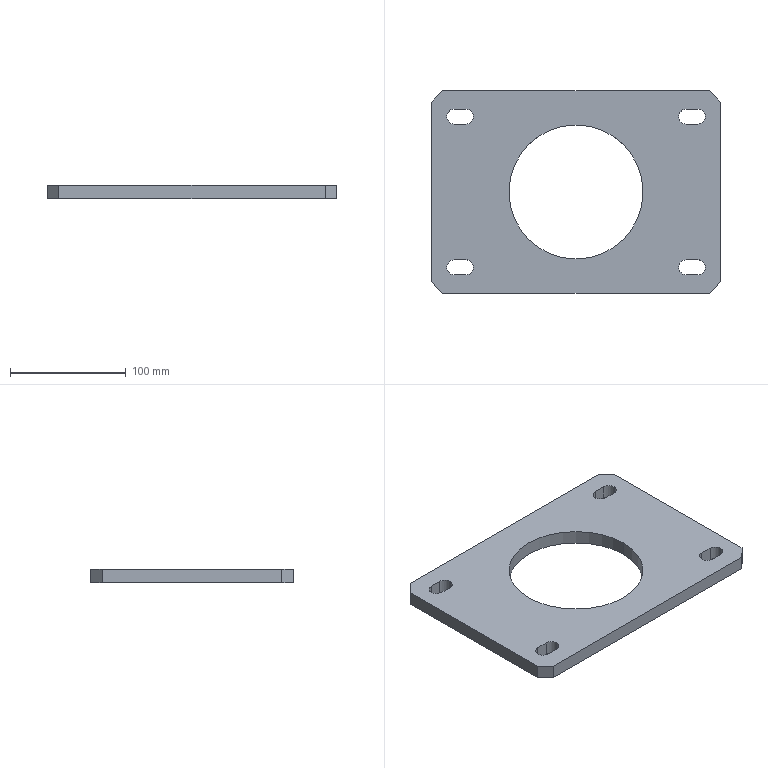Component | SolidWorks | PlanetaryReducer-PLF142Mount1-1 | 1 solid | 32 faces | box 250 x 175 x 12 mm | volume 384260 mm3 | plane 18 | cylinder 14 | commonest cylinder face diameters 13 x12 115.5 x2
build123d program:
from build123d import *

# Parameters (mm, degrees)
SKETCH1_W           = 250
SKETCH1_H           = 175
BOSS_EXTRUDE1_DEPTH = 12
SKETCH2_R           = 57.75
CUT_EXTRUDE1_DEPTH  = 154.053
CHAMFER1_SIZE       = 10
CUT_EXTRUDE2_DEPTH  = 154.053


with BuildPart() as part:
    # Sketch1 → Boss-Extrude1 (new body)
    with BuildSketch(Plane.XY):
        Rectangle(SKETCH1_W, SKETCH1_H)
    extrude(amount=BOSS_EXTRUDE1_DEPTH)

    # Sketch2 → Cut-Extrude1 (cut, through all)
    with BuildSketch(Plane.XY.offset(12)):
        Circle(SKETCH2_R)
    extrude(amount=-CUT_EXTRUDE1_DEPTH, mode=Mode.SUBTRACT)

    # Chamfer1
    chamfer1_edges = [part.edges().sort_by_distance(p)[0] for p in [
        (125, -87.5, 6),
        (-125, -87.5, 6),
        (-125, 87.5, 6),
        (125, 87.5, 6),
    ]]
    chamfer(chamfer1_edges, length=CHAMFER1_SIZE)

    # Sketch3 → Cut-Extrude2 (cut, through all)
    with BuildSketch(Plane.XY.offset(12)):
        with BuildLine():
            Line((-105, 71.5), (-95, 71.5))
            ThreePointArc((-95, 71.5), (-88.5, 65), (-95, 58.5))
            Line((-95, 58.5), (-105, 58.5))
            ThreePointArc((-105, 58.5), (-111.5, 65), (-105, 71.5))
        make_face()
        with BuildLine():
            Line((-105, -58.5), (-95, -58.5))
            ThreePointArc((-95, -58.5), (-88.5, -65), (-95, -71.5))
            Line((-95, -71.5), (-105, -71.5))
            ThreePointArc((-105, -71.5), (-111.5, -65), (-105, -58.5))
        make_face()
        with BuildLine():
            Line((95, -58.5), (105, -58.5))
            ThreePointArc((105, -58.5), (111.5, -65), (105, -71.5))
            Line((105, -71.5), (95, -71.5))
            ThreePointArc((95, -71.5), (88.5, -65), (95, -58.5))
        make_face()
        with BuildLine():
            Line((95, 71.5), (105, 71.5))
            ThreePointArc((105, 71.5), (111.5, 65), (105, 58.5))
            Line((105, 58.5), (95, 58.5))
            ThreePointArc((95, 58.5), (88.5, 65), (95, 71.5))
        make_face()
    extrude(amount=-CUT_EXTRUDE2_DEPTH, mode=Mode.SUBTRACT)


solid = part.part

# Placed as in the assembly
solid = solid.moved(Location((-85, 178, 110), (0, 0, 0)))
STEP:
#1=COLOUR_RGB('',0.7922,0.8196,0.9333);
#2=FILL_AREA_STYLE_COLOUR('',#1);
#3=FILL_AREA_STYLE('',(#2));
#4=SURFACE_STYLE_FILL_AREA(#3);
#5=SURFACE_SIDE_STYLE('',(#4));
#6=SURFACE_STYLE_USAGE(.BOTH.,#5);
#7=PRESENTATION_STYLE_ASSIGNMENT((#6));
#8=CARTESIAN_POINT('',(1.043,9.567,4.331));
#9=VERTEX_POINT('',#8);
#10=CARTESIAN_POINT('',(0.7874,9.823,4.331));
#11=VERTEX_POINT('',#10);
#12=CARTESIAN_POINT('',(0.7874,9.567,4.331));
#13=DIRECTION('',(0.,0.,1.));
#14=DIRECTION('',(1.,0.,0.));
#15=AXIS2_PLACEMENT_3D('',#12,#13,#14);
#16=CIRCLE('',#15,0.2559);
#17=EDGE_CURVE('',#9,#11,#16,.T.);
#18=ORIENTED_EDGE('',*,*,#17,.F.);
#19=CARTESIAN_POINT('',(1.043,9.567,4.803));
#20=VERTEX_POINT('',#19);
#21=CARTESIAN_POINT('',(1.043,9.567,4.331));
#22=DIRECTION('',(0.,0.,1.));
#23=VECTOR('',#22,39.37);
#24=LINE('',#21,#23);
#25=EDGE_CURVE('',#9,#20,#24,.T.);
#26=ORIENTED_EDGE('',*,*,#25,.T.);
#27=CARTESIAN_POINT('',(0.7874,9.823,4.803));
#28=VERTEX_POINT('',#27);
#29=CARTESIAN_POINT('',(0.7874,9.567,4.803));
#30=DIRECTION('',(0.,0.,1.));
#31=DIRECTION('',(1.,0.,0.));
#32=AXIS2_PLACEMENT_3D('',#29,#30,#31);
#33=CIRCLE('',#32,0.2559);
#34=EDGE_CURVE('',#20,#28,#33,.T.);
#35=ORIENTED_EDGE('',*,*,#34,.T.);
#36=CARTESIAN_POINT('',(0.7874,9.823,4.331));
#37=DIRECTION('',(0.,0.,1.));
#38=VECTOR('',#37,39.37);
#39=LINE('',#36,#38);
#40=EDGE_CURVE('',#11,#28,#39,.T.);
#41=ORIENTED_EDGE('',*,*,#40,.F.);
#42=EDGE_LOOP('',(#18,#26,#35,#41));
#43=FACE_OUTER_BOUND('',#42,.T.);
#44=CARTESIAN_POINT('',(0.7874,9.567,4.331));
#45=DIRECTION('',(0.,0.,1.));
#46=DIRECTION('',(1.,0.,0.));
#47=AXIS2_PLACEMENT_3D('',#44,#45,#46);
#48=CYLINDRICAL_SURFACE('',#47,0.2559);
#49=ADVANCED_FACE('',(#43),#48,.F.);
#50=CARTESIAN_POINT('',(1.043,4.449,4.331));
#51=VERTEX_POINT('',#50);
#52=CARTESIAN_POINT('',(0.7874,4.705,4.331));
#53=VERTEX_POINT('',#52);
#54=CARTESIAN_POINT('',(0.7874,4.449,4.331));
#55=DIRECTION('',(0.,0.,1.));
#56=DIRECTION('',(1.,0.,0.));
#57=AXIS2_PLACEMENT_3D('',#54,#55,#56);
#58=CIRCLE('',#57,0.2559);
#59=EDGE_CURVE('',#51,#53,#58,.T.);
#60=ORIENTED_EDGE('',*,*,#59,.F.);
#61=CARTESIAN_POINT('',(1.043,4.449,4.803));
#62=VERTEX_POINT('',#61);
#63=CARTESIAN_POINT('',(1.043,4.449,4.331));
#64=DIRECTION('',(0.,0.,1.));
#65=VECTOR('',#64,39.37);
#66=LINE('',#63,#65);
#67=EDGE_CURVE('',#51,#62,#66,.T.);
#68=ORIENTED_EDGE('',*,*,#67,.T.);
#69=CARTESIAN_POINT('',(0.7874,4.705,4.803));
#70=VERTEX_POINT('',#69);
#71=CARTESIAN_POINT('',(0.7874,4.449,4.803));
#72=DIRECTION('',(0.,0.,1.));
#73=DIRECTION('',(1.,0.,0.));
#74=AXIS2_PLACEMENT_3D('',#71,#72,#73);
#75=CIRCLE('',#74,0.2559);
#76=EDGE_CURVE('',#62,#70,#75,.T.);
#77=ORIENTED_EDGE('',*,*,#76,.T.);
#78=CARTESIAN_POINT('',(0.7874,4.705,4.331));
#79=DIRECTION('',(0.,0.,1.));
#80=VECTOR('',#79,39.37);
#81=LINE('',#78,#80);
#82=EDGE_CURVE('',#53,#70,#81,.T.);
#83=ORIENTED_EDGE('',*,*,#82,.F.);
#84=EDGE_LOOP('',(#60,#68,#77,#83));
#85=FACE_OUTER_BOUND('',#84,.T.);
#86=CARTESIAN_POINT('',(0.7874,4.449,4.331));
#87=DIRECTION('',(0.,0.,1.));
#88=DIRECTION('',(1.,0.,0.));
#89=AXIS2_PLACEMENT_3D('',#86,#87,#88);
#90=CYLINDRICAL_SURFACE('',#89,0.2559);
#91=ADVANCED_FACE('',(#85),#90,.F.);
#92=CARTESIAN_POINT('',(-6.831,4.449,4.331));
#93=VERTEX_POINT('',#92);
#94=CARTESIAN_POINT('',(-7.087,4.705,4.331));
#95=VERTEX_POINT('',#94);
#96=CARTESIAN_POINT('',(-7.087,4.449,4.331));
#97=DIRECTION('',(0.,0.,1.));
#98=DIRECTION('',(1.,0.,0.));
#99=AXIS2_PLACEMENT_3D('',#96,#97,#98);
#100=CIRCLE('',#99,0.2559);
#101=EDGE_CURVE('',#93,#95,#100,.T.);
#102=ORIENTED_EDGE('',*,*,#101,.F.);
#103=CARTESIAN_POINT('',(-6.831,4.449,4.803));
#104=VERTEX_POINT('',#103);
#105=CARTESIAN_POINT('',(-6.831,4.449,4.331));
#106=DIRECTION('',(0.,0.,1.));
#107=VECTOR('',#106,39.37);
#108=LINE('',#105,#107);
#109=EDGE_CURVE('',#93,#104,#108,.T.);
#110=ORIENTED_EDGE('',*,*,#109,.T.);
#111=CARTESIAN_POINT('',(-7.087,4.705,4.803));
#112=VERTEX_POINT('',#111);
#113=CARTESIAN_POINT('',(-7.087,4.449,4.803));
#114=DIRECTION('',(0.,0.,1.));
#115=DIRECTION('',(1.,0.,0.));
#116=AXIS2_PLACEMENT_3D('',#113,#114,#115);
#117=CIRCLE('',#116,0.2559);
#118=EDGE_CURVE('',#104,#112,#117,.T.);
#119=ORIENTED_EDGE('',*,*,#118,.T.);
#120=CARTESIAN_POINT('',(-7.087,4.705,4.331));
#121=DIRECTION('',(0.,0.,1.));
#122=VECTOR('',#121,39.37);
#123=LINE('',#120,#122);
#124=EDGE_CURVE('',#95,#112,#123,.T.);
#125=ORIENTED_EDGE('',*,*,#124,.F.);
#126=EDGE_LOOP('',(#102,#110,#119,#125));
#127=FACE_OUTER_BOUND('',#126,.T.);
#128=CARTESIAN_POINT('',(-7.087,4.449,4.331));
#129=DIRECTION('',(0.,0.,1.));
#130=DIRECTION('',(1.,0.,0.));
#131=AXIS2_PLACEMENT_3D('',#128,#129,#130);
#132=CYLINDRICAL_SURFACE('',#131,0.2559);
#133=ADVANCED_FACE('',(#127),#132,.F.);
#134=CARTESIAN_POINT('',(-6.831,9.567,4.331));
#135=VERTEX_POINT('',#134);
#136=CARTESIAN_POINT('',(-7.087,9.823,4.331));
#137=VERTEX_POINT('',#136);
#138=CARTESIAN_POINT('',(-7.087,9.567,4.331));
#139=DIRECTION('',(0.,0.,1.));
#140=DIRECTION('',(1.,0.,0.));
#141=AXIS2_PLACEMENT_3D('',#138,#139,#140);
#142=CIRCLE('',#141,0.2559);
#143=EDGE_CURVE('',#135,#137,#142,.T.);
#144=ORIENTED_EDGE('',*,*,#143,.F.);
#145=CARTESIAN_POINT('',(-6.831,9.567,4.803));
#146=VERTEX_POINT('',#145);
#147=CARTESIAN_POINT('',(-6.831,9.567,4.331));
#148=DIRECTION('',(0.,0.,1.));
#149=VECTOR('',#148,39.37);
#150=LINE('',#147,#149);
#151=EDGE_CURVE('',#135,#146,#150,.T.);
#152=ORIENTED_EDGE('',*,*,#151,.T.);
#153=CARTESIAN_POINT('',(-7.087,9.823,4.803));
#154=VERTEX_POINT('',#153);
#155=CARTESIAN_POINT('',(-7.087,9.567,4.803));
#156=DIRECTION('',(0.,0.,1.));
#157=DIRECTION('',(1.,0.,0.));
#158=AXIS2_PLACEMENT_3D('',#155,#156,#157);
#159=CIRCLE('',#158,0.2559);
#160=EDGE_CURVE('',#146,#154,#159,.T.);
#161=ORIENTED_EDGE('',*,*,#160,.T.);
#162=CARTESIAN_POINT('',(-7.087,9.823,4.331));
#163=DIRECTION('',(0.,0.,1.));
#164=VECTOR('',#163,39.37);
#165=LINE('',#162,#164);
#166=EDGE_CURVE('',#137,#154,#165,.T.);
#167=ORIENTED_EDGE('',*,*,#166,.F.);
#168=EDGE_LOOP('',(#144,#152,#161,#167));
#169=FACE_OUTER_BOUND('',#168,.T.);
#170=CARTESIAN_POINT('',(-7.087,9.567,4.331));
#171=DIRECTION('',(0.,0.,1.));
#172=DIRECTION('',(1.,0.,0.));
#173=AXIS2_PLACEMENT_3D('',#170,#171,#172);
#174=CYLINDRICAL_SURFACE('',#173,0.2559);
#175=ADVANCED_FACE('',(#169),#174,.F.);
#176=CARTESIAN_POINT('',(-5.62,7.008,4.331));
#177=VERTEX_POINT('',#176);
#178=CARTESIAN_POINT('',(-1.073,7.008,4.331));
#179=VERTEX_POINT('',#178);
#180=CARTESIAN_POINT('',(-3.346,7.008,4.331));
#181=DIRECTION('',(0.,0.,1.));
#182=DIRECTION('',(1.,0.,0.));
#183=AXIS2_PLACEMENT_3D('',#180,#181,#182);
#184=CIRCLE('',#183,2.274);
#185=EDGE_CURVE('',#177,#179,#184,.T.);
#186=ORIENTED_EDGE('',*,*,#185,.F.);
#187=CARTESIAN_POINT('',(-5.62,7.008,4.803));
#188=VERTEX_POINT('',#187);
#189=CARTESIAN_POINT('',(-5.62,7.008,4.331));
#190=DIRECTION('',(0.,0.,1.));
#191=VECTOR('',#190,39.37);
#192=LINE('',#189,#191);
#193=EDGE_CURVE('',#177,#188,#192,.T.);
#194=ORIENTED_EDGE('',*,*,#193,.T.);
#195=CARTESIAN_POINT('',(-1.073,7.008,4.803));
#196=VERTEX_POINT('',#195);
#197=CARTESIAN_POINT('',(-3.346,7.008,4.803));
#198=DIRECTION('',(0.,0.,1.));
#199=DIRECTION('',(1.,0.,0.));
#200=AXIS2_PLACEMENT_3D('',#197,#198,#199);
#201=CIRCLE('',#200,2.274);
#202=EDGE_CURVE('',#188,#196,#201,.T.);
#203=ORIENTED_EDGE('',*,*,#202,.T.);
#204=CARTESIAN_POINT('',(-1.073,7.008,4.331));
#205=DIRECTION('',(0.,0.,1.));
#206=VECTOR('',#205,39.37);
#207=LINE('',#204,#206);
#208=EDGE_CURVE('',#179,#196,#207,.T.);
#209=ORIENTED_EDGE('',*,*,#208,.F.);
#210=EDGE_LOOP('',(#186,#194,#203,#209));
#211=FACE_OUTER_BOUND('',#210,.T.);
#212=CARTESIAN_POINT('',(-3.346,7.008,4.331));
#213=DIRECTION('',(0.,0.,1.));
#214=DIRECTION('',(1.,0.,0.));
#215=AXIS2_PLACEMENT_3D('',#212,#213,#214);
#216=CYLINDRICAL_SURFACE('',#215,2.274);
#217=ADVANCED_FACE('',(#211),#216,.F.);
#218=CARTESIAN_POINT('',(1.575,3.957,4.803));
#219=VERTEX_POINT('',#218);
#220=CARTESIAN_POINT('',(1.575,10.059,4.803));
#221=VERTEX_POINT('',#220);
#222=CARTESIAN_POINT('',(1.575,10.453,4.803));
#223=DIRECTION('',(-0.,1.,0.));
#224=VECTOR('',#223,39.37);
#225=LINE('',#222,#224);
#226=EDGE_CURVE('',#219,#221,#225,.T.);
#227=ORIENTED_EDGE('',*,*,#226,.F.);
#228=CARTESIAN_POINT('',(1.575,3.957,4.331));
#229=VERTEX_POINT('',#228);
#230=CARTESIAN_POINT('',(1.575,3.957,4.803));
#231=DIRECTION('',(0.,0.,-1.));
#232=VECTOR('',#231,39.37);
#233=LINE('',#230,#232);
#234=EDGE_CURVE('',#219,#229,#233,.T.);
#235=ORIENTED_EDGE('',*,*,#234,.T.);
#236=CARTESIAN_POINT('',(1.575,10.059,4.331));
#237=VERTEX_POINT('',#236);
#238=CARTESIAN_POINT('',(1.575,10.453,4.331));
#239=DIRECTION('',(-0.,1.,0.));
#240=VECTOR('',#239,39.37);
#241=LINE('',#238,#240);
#242=EDGE_CURVE('',#229,#237,#241,.T.);
#243=ORIENTED_EDGE('',*,*,#242,.T.);
#244=CARTESIAN_POINT('',(1.575,10.059,4.803));
#245=DIRECTION('',(0.,0.,1.));
#246=VECTOR('',#245,39.37);
#247=LINE('',#244,#246);
#248=EDGE_CURVE('',#237,#221,#247,.T.);
#249=ORIENTED_EDGE('',*,*,#248,.T.);
#250=EDGE_LOOP('',(#227,#235,#243,#249));
#251=FACE_OUTER_BOUND('',#250,.T.);
#252=CARTESIAN_POINT('',(1.575,10.453,4.803));
#253=DIRECTION('',(-1.,-0.,0.));
#254=DIRECTION('',(0.,-1.,0.));
#255=AXIS2_PLACEMENT_3D('',#252,#253,#254);
#256=PLANE('',#255);
#257=ADVANCED_FACE('',(#251),#256,.F.);
#258=CARTESIAN_POINT('',(1.181,10.453,4.331));
#259=VERTEX_POINT('',#258);
#260=CARTESIAN_POINT('',(-7.874,10.453,4.331));
#261=VERTEX_POINT('',#260);
#262=CARTESIAN_POINT('',(-8.268,10.453,4.331));
#263=DIRECTION('',(-1.,0.,0.));
#264=VECTOR('',#263,39.37);
#265=LINE('',#262,#264);
#266=EDGE_CURVE('',#259,#261,#265,.T.);
#267=ORIENTED_EDGE('',*,*,#266,.T.);
#268=CARTESIAN_POINT('',(-7.874,10.453,4.803));
#269=VERTEX_POINT('',#268);
#270=CARTESIAN_POINT('',(-7.874,10.453,4.803));
#271=DIRECTION('',(0.,0.,1.));
#272=VECTOR('',#271,39.37);
#273=LINE('',#270,#272);
#274=EDGE_CURVE('',#261,#269,#273,.T.);
#275=ORIENTED_EDGE('',*,*,#274,.T.);
#276=CARTESIAN_POINT('',(1.181,10.453,4.803));
#277=VERTEX_POINT('',#276);
#278=CARTESIAN_POINT('',(-8.268,10.453,4.803));
#279=DIRECTION('',(-1.,0.,0.));
#280=VECTOR('',#279,39.37);
#281=LINE('',#278,#280);
#282=EDGE_CURVE('',#277,#269,#281,.T.);
#283=ORIENTED_EDGE('',*,*,#282,.F.);
#284=CARTESIAN_POINT('',(1.181,10.453,4.803));
#285=DIRECTION('',(0.,0.,-1.));
#286=VECTOR('',#285,39.37);
#287=LINE('',#284,#286);
#288=EDGE_CURVE('',#277,#259,#287,.T.);
#289=ORIENTED_EDGE('',*,*,#288,.T.);
#290=EDGE_LOOP('',(#267,#275,#283,#289));
#291=FACE_OUTER_BOUND('',#290,.T.);
#292=CARTESIAN_POINT('',(-8.268,10.453,4.803));
#293=DIRECTION('',(0.,-1.,0.));
#294=DIRECTION('',(0.,0.,-1.));
#295=AXIS2_PLACEMENT_3D('',#292,#293,#294);
#296=PLANE('',#295);
#297=ADVANCED_FACE('',(#291),#296,.F.);
#298=CARTESIAN_POINT('',(-8.268,10.059,4.331));
#299=VERTEX_POINT('',#298);
#300=CARTESIAN_POINT('',(-8.268,3.957,4.331));
#301=VERTEX_POINT('',#300);
#302=CARTESIAN_POINT('',(-8.268,10.453,4.331));
#303=DIRECTION('',(0.,-1.,0.));
#304=VECTOR('',#303,39.37);
#305=LINE('',#302,#304);
#306=EDGE_CURVE('',#299,#301,#305,.T.);
#307=ORIENTED_EDGE('',*,*,#306,.T.);
#308=CARTESIAN_POINT('',(-8.268,3.957,4.803));
#309=VERTEX_POINT('',#308);
#310=CARTESIAN_POINT('',(-8.268,3.957,4.803));
#311=DIRECTION('',(0.,0.,1.));
#312=VECTOR('',#311,39.37);
#313=LINE('',#310,#312);
#314=EDGE_CURVE('',#301,#309,#313,.T.);
#315=ORIENTED_EDGE('',*,*,#314,.T.);
#316=CARTESIAN_POINT('',(-8.268,10.059,4.803));
#317=VERTEX_POINT('',#316);
#318=CARTESIAN_POINT('',(-8.268,10.453,4.803));
#319=DIRECTION('',(0.,-1.,0.));
#320=VECTOR('',#319,39.37);
#321=LINE('',#318,#320);
#322=EDGE_CURVE('',#317,#309,#321,.T.);
#323=ORIENTED_EDGE('',*,*,#322,.F.);
#324=CARTESIAN_POINT('',(-8.268,10.059,4.803));
#325=DIRECTION('',(0.,0.,-1.));
#326=VECTOR('',#325,39.37);
#327=LINE('',#324,#326);
#328=EDGE_CURVE('',#317,#299,#327,.T.);
#329=ORIENTED_EDGE('',*,*,#328,.T.);
#330=EDGE_LOOP('',(#307,#315,#323,#329));
#331=FACE_OUTER_BOUND('',#330,.T.);
#332=CARTESIAN_POINT('',(-8.268,10.453,4.803));
#333=DIRECTION('',(1.,0.,0.));
#334=DIRECTION('',(-0.,1.,0.));
#335=AXIS2_PLACEMENT_3D('',#332,#333,#334);
#336=PLANE('',#335);
#337=ADVANCED_FACE('',(#331),#336,.F.);
#338=CARTESIAN_POINT('',(-7.874,3.563,4.331));
#339=VERTEX_POINT('',#338);
#340=CARTESIAN_POINT('',(1.181,3.563,4.331));
#341=VERTEX_POINT('',#340);
#342=CARTESIAN_POINT('',(-8.268,3.563,4.331));
#343=DIRECTION('',(1.,0.,0.));
#344=VECTOR('',#343,39.37);
#345=LINE('',#342,#344);
#346=EDGE_CURVE('',#339,#341,#345,.T.);
#347=ORIENTED_EDGE('',*,*,#346,.T.);
#348=CARTESIAN_POINT('',(1.181,3.563,4.803));
#349=VERTEX_POINT('',#348);
#350=CARTESIAN_POINT('',(1.181,3.563,4.803));
#351=DIRECTION('',(0.,0.,1.));
#352=VECTOR('',#351,39.37);
#353=LINE('',#350,#352);
#354=EDGE_CURVE('',#341,#349,#353,.T.);
#355=ORIENTED_EDGE('',*,*,#354,.T.);
#356=CARTESIAN_POINT('',(-7.874,3.563,4.803));
#357=VERTEX_POINT('',#356);
#358=CARTESIAN_POINT('',(-8.268,3.563,4.803));
#359=DIRECTION('',(1.,0.,0.));
#360=VECTOR('',#359,39.37);
#361=LINE('',#358,#360);
#362=EDGE_CURVE('',#357,#349,#361,.T.);
#363=ORIENTED_EDGE('',*,*,#362,.F.);
#364=CARTESIAN_POINT('',(-7.874,3.563,4.803));
#365=DIRECTION('',(0.,0.,-1.));
#366=VECTOR('',#365,39.37);
#367=LINE('',#364,#366);
#368=EDGE_CURVE('',#357,#339,#367,.T.);
#369=ORIENTED_EDGE('',*,*,#368,.T.);
#370=EDGE_LOOP('',(#347,#355,#363,#369));
#371=FACE_OUTER_BOUND('',#370,.T.);
#372=CARTESIAN_POINT('',(-8.268,3.563,4.803));
#373=DIRECTION('',(0.,1.,0.));
#374=DIRECTION('',(0.,0.,1.));
#375=AXIS2_PLACEMENT_3D('',#372,#373,#374);
#376=PLANE('',#375);
#377=ADVANCED_FACE('',(#371),#376,.F.);
#378=CARTESIAN_POINT('',(0.3937,9.823,4.803));
#379=VERTEX_POINT('',#378);
#380=CARTESIAN_POINT('',(0.3937,9.311,4.803));
#381=VERTEX_POINT('',#380);
#382=CARTESIAN_POINT('',(0.3937,9.567,4.803));
#383=DIRECTION('',(0.,0.,1.));
#384=DIRECTION('',(1.,0.,0.));
#385=AXIS2_PLACEMENT_3D('',#382,#383,#384);
#386=CIRCLE('',#385,0.2559);
#387=EDGE_CURVE('',#379,#381,#386,.T.);
#388=ORIENTED_EDGE('',*,*,#387,.F.);
#389=CARTESIAN_POINT('',(0.3937,9.823,4.803));
#390=DIRECTION('',(-1.,0.,0.));
#391=VECTOR('',#390,39.37);
#392=LINE('',#389,#391);
#393=EDGE_CURVE('',#28,#379,#392,.T.);
#394=ORIENTED_EDGE('',*,*,#393,.F.);
#395=ORIENTED_EDGE('',*,*,#34,.F.);
#396=CARTESIAN_POINT('',(0.7874,9.311,4.803));
#397=VERTEX_POINT('',#396);
#398=CARTESIAN_POINT('',(0.7874,9.567,4.803));
#399=DIRECTION('',(0.,0.,1.));
#400=DIRECTION('',(1.,0.,0.));
#401=AXIS2_PLACEMENT_3D('',#398,#399,#400);
#402=CIRCLE('',#401,0.2559);
#403=EDGE_CURVE('',#397,#20,#402,.T.);
#404=ORIENTED_EDGE('',*,*,#403,.F.);
#405=CARTESIAN_POINT('',(0.3937,9.311,4.803));
#406=DIRECTION('',(1.,0.,0.));
#407=VECTOR('',#406,39.37);
#408=LINE('',#405,#407);
#409=EDGE_CURVE('',#381,#397,#408,.T.);
#410=ORIENTED_EDGE('',*,*,#409,.F.);
#411=EDGE_LOOP('',(#388,#394,#395,#404,#410));
#412=FACE_BOUND('',#411,.T.);
#413=CARTESIAN_POINT('',(0.3937,4.705,4.803));
#414=VERTEX_POINT('',#413);
#415=CARTESIAN_POINT('',(0.3937,4.193,4.803));
#416=VERTEX_POINT('',#415);
#417=CARTESIAN_POINT('',(0.3937,4.449,4.803));
#418=DIRECTION('',(0.,0.,1.));
#419=DIRECTION('',(1.,0.,0.));
#420=AXIS2_PLACEMENT_3D('',#417,#418,#419);
#421=CIRCLE('',#420,0.2559);
#422=EDGE_CURVE('',#414,#416,#421,.T.);
#423=ORIENTED_EDGE('',*,*,#422,.F.);
#424=CARTESIAN_POINT('',(0.3937,4.705,4.803));
#425=DIRECTION('',(-1.,0.,0.));
#426=VECTOR('',#425,39.37);
#427=LINE('',#424,#426);
#428=EDGE_CURVE('',#70,#414,#427,.T.);
#429=ORIENTED_EDGE('',*,*,#428,.F.);
#430=ORIENTED_EDGE('',*,*,#76,.F.);
#431=CARTESIAN_POINT('',(0.7874,4.193,4.803));
#432=VERTEX_POINT('',#431);
#433=CARTESIAN_POINT('',(0.7874,4.449,4.803));
#434=DIRECTION('',(0.,0.,1.));
#435=DIRECTION('',(1.,0.,0.));
#436=AXIS2_PLACEMENT_3D('',#433,#434,#435);
#437=CIRCLE('',#436,0.2559);
#438=EDGE_CURVE('',#432,#62,#437,.T.);
#439=ORIENTED_EDGE('',*,*,#438,.F.);
#440=CARTESIAN_POINT('',(0.3937,4.193,4.803));
#441=DIRECTION('',(1.,0.,0.));
#442=VECTOR('',#441,39.37);
#443=LINE('',#440,#442);
#444=EDGE_CURVE('',#416,#432,#443,.T.);
#445=ORIENTED_EDGE('',*,*,#444,.F.);
#446=EDGE_LOOP('',(#423,#429,#430,#439,#445));
#447=FACE_BOUND('',#446,.T.);
#448=CARTESIAN_POINT('',(-7.48,4.705,4.803));
#449=VERTEX_POINT('',#448);
#450=CARTESIAN_POINT('',(-7.48,4.193,4.803));
#451=VERTEX_POINT('',#450);
#452=CARTESIAN_POINT('',(-7.48,4.449,4.803));
#453=DIRECTION('',(0.,0.,1.));
#454=DIRECTION('',(1.,0.,0.));
#455=AXIS2_PLACEMENT_3D('',#452,#453,#454);
#456=CIRCLE('',#455,0.2559);
#457=EDGE_CURVE('',#449,#451,#456,.T.);
#458=ORIENTED_EDGE('',*,*,#457,.F.);
#459=CARTESIAN_POINT('',(-7.48,4.705,4.803));
#460=DIRECTION('',(-1.,0.,0.));
#461=VECTOR('',#460,39.37);
#462=LINE('',#459,#461);
#463=EDGE_CURVE('',#112,#449,#462,.T.);
#464=ORIENTED_EDGE('',*,*,#463,.F.);
#465=ORIENTED_EDGE('',*,*,#118,.F.);
#466=CARTESIAN_POINT('',(-7.087,4.193,4.803));
#467=VERTEX_POINT('',#466);
#468=CARTESIAN_POINT('',(-7.087,4.449,4.803));
#469=DIRECTION('',(0.,0.,1.));
#470=DIRECTION('',(1.,0.,0.));
#471=AXIS2_PLACEMENT_3D('',#468,#469,#470);
#472=CIRCLE('',#471,0.2559);
#473=EDGE_CURVE('',#467,#104,#472,.T.);
#474=ORIENTED_EDGE('',*,*,#473,.F.);
#475=CARTESIAN_POINT('',(-7.48,4.193,4.803));
#476=DIRECTION('',(1.,0.,0.));
#477=VECTOR('',#476,39.37);
#478=LINE('',#475,#477);
#479=EDGE_CURVE('',#451,#467,#478,.T.);
#480=ORIENTED_EDGE('',*,*,#479,.F.);
#481=EDGE_LOOP('',(#458,#464,#465,#474,#480));
#482=FACE_BOUND('',#481,.T.);
#483=CARTESIAN_POINT('',(-7.48,9.823,4.803));
#484=VERTEX_POINT('',#483);
#485=CARTESIAN_POINT('',(-7.48,9.311,4.803));
#486=VERTEX_POINT('',#485);
#487=CARTESIAN_POINT('',(-7.48,9.567,4.803));
#488=DIRECTION('',(0.,0.,1.));
#489=DIRECTION('',(1.,0.,0.));
#490=AXIS2_PLACEMENT_3D('',#487,#488,#489);
#491=CIRCLE('',#490,0.2559);
#492=EDGE_CURVE('',#484,#486,#491,.T.);
#493=ORIENTED_EDGE('',*,*,#492,.F.);
#494=CARTESIAN_POINT('',(-7.48,9.823,4.803));
#495=DIRECTION('',(-1.,0.,0.));
#496=VECTOR('',#495,39.37);
#497=LINE('',#494,#496);
#498=EDGE_CURVE('',#154,#484,#497,.T.);
#499=ORIENTED_EDGE('',*,*,#498,.F.);
#500=ORIENTED_EDGE('',*,*,#160,.F.);
#501=CARTESIAN_POINT('',(-7.087,9.311,4.803));
#502=VERTEX_POINT('',#501);
#503=CARTESIAN_POINT('',(-7.087,9.567,4.803));
#504=DIRECTION('',(0.,0.,1.));
#505=DIRECTION('',(1.,0.,0.));
#506=AXIS2_PLACEMENT_3D('',#503,#504,#505);
#507=CIRCLE('',#506,0.2559);
#508=EDGE_CURVE('',#502,#146,#507,.T.);
#509=ORIENTED_EDGE('',*,*,#508,.F.);
#510=CARTESIAN_POINT('',(-7.48,9.311,4.803));
#511=DIRECTION('',(1.,0.,0.));
#512=VECTOR('',#511,39.37);
#513=LINE('',#510,#512);
#514=EDGE_CURVE('',#486,#502,#513,.T.);
#515=ORIENTED_EDGE('',*,*,#514,.F.);
#516=EDGE_LOOP('',(#493,#499,#500,#509,#515));
#517=FACE_BOUND('',#516,.T.);
#518=CARTESIAN_POINT('',(-3.346,7.008,4.803));
#519=DIRECTION('',(0.,0.,1.));
#520=DIRECTION('',(1.,0.,0.));
#521=AXIS2_PLACEMENT_3D('',#518,#519,#520);
#522=CIRCLE('',#521,2.274);
#523=EDGE_CURVE('',#196,#188,#522,.T.);
#524=ORIENTED_EDGE('',*,*,#523,.F.);
#525=ORIENTED_EDGE('',*,*,#202,.F.);
#526=EDGE_LOOP('',(#524,#525));
#527=FACE_BOUND('',#526,.T.);
#528=ORIENTED_EDGE('',*,*,#362,.T.);
#529=CARTESIAN_POINT('',(0.6398,3.022,4.803));
#530=DIRECTION('',(0.7071,0.7071,0.));
#531=VECTOR('',#530,39.37);
#532=LINE('',#529,#531);
#533=EDGE_CURVE('',#349,#219,#532,.T.);
#534=ORIENTED_EDGE('',*,*,#533,.T.);
#535=ORIENTED_EDGE('',*,*,#226,.T.);
#536=CARTESIAN_POINT('',(0.6398,10.994,4.803));
#537=DIRECTION('',(-0.7071,0.7071,0.));
#538=VECTOR('',#537,39.37);
#539=LINE('',#536,#538);
#540=EDGE_CURVE('',#221,#277,#539,.T.);
#541=ORIENTED_EDGE('',*,*,#540,.T.);
#542=ORIENTED_EDGE('',*,*,#282,.T.);
#543=CARTESIAN_POINT('',(-7.333,10.994,4.803));
#544=DIRECTION('',(-0.7071,-0.7071,0.));
#545=VECTOR('',#544,39.37);
#546=LINE('',#543,#545);
#547=EDGE_CURVE('',#269,#317,#546,.T.);
#548=ORIENTED_EDGE('',*,*,#547,.T.);
#549=ORIENTED_EDGE('',*,*,#322,.T.);
#550=CARTESIAN_POINT('',(-7.333,3.022,4.803));
#551=DIRECTION('',(0.7071,-0.7071,0.));
#552=VECTOR('',#551,39.37);
#553=LINE('',#550,#552);
#554=EDGE_CURVE('',#309,#357,#553,.T.);
#555=ORIENTED_EDGE('',*,*,#554,.T.);
#556=EDGE_LOOP('',(#528,#534,#535,#541,#542,#548,#549,#555));
#557=FACE_OUTER_BOUND('',#556,.T.);
#558=CARTESIAN_POINT('',(-3.346,7.008,4.803));
#559=DIRECTION('',(0.,0.,1.));
#560=DIRECTION('',(1.,0.,0.));
#561=AXIS2_PLACEMENT_3D('',#558,#559,#560);
#562=PLANE('',#561);
#563=ADVANCED_FACE('',(#412,#447,#482,#517,#527,#557),#562,.T.);
#564=CARTESIAN_POINT('',(0.3937,9.823,4.331));
#565=VERTEX_POINT('',#564);
#566=CARTESIAN_POINT('',(0.3937,9.823,4.331));
#567=DIRECTION('',(-1.,0.,0.));
#568=VECTOR('',#567,39.37);
#569=LINE('',#566,#568);
#570=EDGE_CURVE('',#11,#565,#569,.T.);
#571=ORIENTED_EDGE('',*,*,#570,.T.);
#572=CARTESIAN_POINT('',(0.3937,9.311,4.331));
#573=VERTEX_POINT('',#572);
#574=CARTESIAN_POINT('',(0.3937,9.567,4.331));
#575=DIRECTION('',(0.,0.,1.));
#576=DIRECTION('',(1.,0.,0.));
#577=AXIS2_PLACEMENT_3D('',#574,#575,#576);
#578=CIRCLE('',#577,0.2559);
#579=EDGE_CURVE('',#565,#573,#578,.T.);
#580=ORIENTED_EDGE('',*,*,#579,.T.);
#581=CARTESIAN_POINT('',(0.7874,9.311,4.331));
#582=VERTEX_POINT('',#581);
#583=CARTESIAN_POINT('',(0.3937,9.311,4.331));
#584=DIRECTION('',(1.,0.,0.));
#585=VECTOR('',#584,39.37);
#586=LINE('',#583,#585);
#587=EDGE_CURVE('',#573,#582,#586,.T.);
#588=ORIENTED_EDGE('',*,*,#587,.T.);
#589=CARTESIAN_POINT('',(0.7874,9.567,4.331));
#590=DIRECTION('',(0.,0.,1.));
#591=DIRECTION('',(1.,0.,0.));
#592=AXIS2_PLACEMENT_3D('',#589,#590,#591);
#593=CIRCLE('',#592,0.2559);
#594=EDGE_CURVE('',#582,#9,#593,.T.);
#595=ORIENTED_EDGE('',*,*,#594,.T.);
#596=ORIENTED_EDGE('',*,*,#17,.T.);
#597=EDGE_LOOP('',(#571,#580,#588,#595,#596));
#598=FACE_BOUND('',#597,.T.);
#599=CARTESIAN_POINT('',(0.3937,4.705,4.331));
#600=VERTEX_POINT('',#599);
#601=CARTESIAN_POINT('',(0.3937,4.705,4.331));
#602=DIRECTION('',(-1.,0.,0.));
#603=VECTOR('',#602,39.37);
#604=LINE('',#601,#603);
#605=EDGE_CURVE('',#53,#600,#604,.T.);
#606=ORIENTED_EDGE('',*,*,#605,.T.);
#607=CARTESIAN_POINT('',(0.3937,4.193,4.331));
#608=VERTEX_POINT('',#607);
#609=CARTESIAN_POINT('',(0.3937,4.449,4.331));
#610=DIRECTION('',(0.,0.,1.));
#611=DIRECTION('',(1.,0.,0.));
#612=AXIS2_PLACEMENT_3D('',#609,#610,#611);
#613=CIRCLE('',#612,0.2559);
#614=EDGE_CURVE('',#600,#608,#613,.T.);
#615=ORIENTED_EDGE('',*,*,#614,.T.);
#616=CARTESIAN_POINT('',(0.7874,4.193,4.331));
#617=VERTEX_POINT('',#616);
#618=CARTESIAN_POINT('',(0.3937,4.193,4.331));
#619=DIRECTION('',(1.,0.,0.));
#620=VECTOR('',#619,39.37);
#621=LINE('',#618,#620);
#622=EDGE_CURVE('',#608,#617,#621,.T.);
#623=ORIENTED_EDGE('',*,*,#622,.T.);
#624=CARTESIAN_POINT('',(0.7874,4.449,4.331));
#625=DIRECTION('',(0.,0.,1.));
#626=DIRECTION('',(1.,0.,0.));
#627=AXIS2_PLACEMENT_3D('',#624,#625,#626);
#628=CIRCLE('',#627,0.2559);
#629=EDGE_CURVE('',#617,#51,#628,.T.);
#630=ORIENTED_EDGE('',*,*,#629,.T.);
#631=ORIENTED_EDGE('',*,*,#59,.T.);
#632=EDGE_LOOP('',(#606,#615,#623,#630,#631));
#633=FACE_BOUND('',#632,.T.);
#634=CARTESIAN_POINT('',(-7.48,4.705,4.331));
#635=VERTEX_POINT('',#634);
#636=CARTESIAN_POINT('',(-7.48,4.705,4.331));
#637=DIRECTION('',(-1.,0.,0.));
#638=VECTOR('',#637,39.37);
#639=LINE('',#636,#638);
#640=EDGE_CURVE('',#95,#635,#639,.T.);
#641=ORIENTED_EDGE('',*,*,#640,.T.);
#642=CARTESIAN_POINT('',(-7.48,4.193,4.331));
#643=VERTEX_POINT('',#642);
#644=CARTESIAN_POINT('',(-7.48,4.449,4.331));
#645=DIRECTION('',(0.,0.,1.));
#646=DIRECTION('',(1.,0.,0.));
#647=AXIS2_PLACEMENT_3D('',#644,#645,#646);
#648=CIRCLE('',#647,0.2559);
#649=EDGE_CURVE('',#635,#643,#648,.T.);
#650=ORIENTED_EDGE('',*,*,#649,.T.);
#651=CARTESIAN_POINT('',(-7.087,4.193,4.331));
#652=VERTEX_POINT('',#651);
#653=CARTESIAN_POINT('',(-7.48,4.193,4.331));
#654=DIRECTION('',(1.,0.,0.));
#655=VECTOR('',#654,39.37);
#656=LINE('',#653,#655);
#657=EDGE_CURVE('',#643,#652,#656,.T.);
#658=ORIENTED_EDGE('',*,*,#657,.T.);
#659=CARTESIAN_POINT('',(-7.087,4.449,4.331));
#660=DIRECTION('',(0.,0.,1.));
#661=DIRECTION('',(1.,0.,0.));
#662=AXIS2_PLACEMENT_3D('',#659,#660,#661);
#663=CIRCLE('',#662,0.2559);
#664=EDGE_CURVE('',#652,#93,#663,.T.);
#665=ORIENTED_EDGE('',*,*,#664,.T.);
#666=ORIENTED_EDGE('',*,*,#101,.T.);
#667=EDGE_LOOP('',(#641,#650,#658,#665,#666));
#668=FACE_BOUND('',#667,.T.);
#669=CARTESIAN_POINT('',(-7.48,9.823,4.331));
#670=VERTEX_POINT('',#669);
#671=CARTESIAN_POINT('',(-7.48,9.823,4.331));
#672=DIRECTION('',(-1.,0.,0.));
#673=VECTOR('',#672,39.37);
#674=LINE('',#671,#673);
#675=EDGE_CURVE('',#137,#670,#674,.T.);
#676=ORIENTED_EDGE('',*,*,#675,.T.);
#677=CARTESIAN_POINT('',(-7.48,9.311,4.331));
#678=VERTEX_POINT('',#677);
#679=CARTESIAN_POINT('',(-7.48,9.567,4.331));
#680=DIRECTION('',(0.,0.,1.));
#681=DIRECTION('',(1.,0.,0.));
#682=AXIS2_PLACEMENT_3D('',#679,#680,#681);
#683=CIRCLE('',#682,0.2559);
#684=EDGE_CURVE('',#670,#678,#683,.T.);
#685=ORIENTED_EDGE('',*,*,#684,.T.);
#686=CARTESIAN_POINT('',(-7.087,9.311,4.331));
#687=VERTEX_POINT('',#686);
#688=CARTESIAN_POINT('',(-7.48,9.311,4.331));
#689=DIRECTION('',(1.,0.,0.));
#690=VECTOR('',#689,39.37);
#691=LINE('',#688,#690);
#692=EDGE_CURVE('',#678,#687,#691,.T.);
#693=ORIENTED_EDGE('',*,*,#692,.T.);
#694=CARTESIAN_POINT('',(-7.087,9.567,4.331));
#695=DIRECTION('',(0.,0.,1.));
#696=DIRECTION('',(1.,0.,0.));
#697=AXIS2_PLACEMENT_3D('',#694,#695,#696);
#698=CIRCLE('',#697,0.2559);
#699=EDGE_CURVE('',#687,#135,#698,.T.);
#700=ORIENTED_EDGE('',*,*,#699,.T.);
#701=ORIENTED_EDGE('',*,*,#143,.T.);
#702=EDGE_LOOP('',(#676,#685,#693,#700,#701));
#703=FACE_BOUND('',#702,.T.);
#704=CARTESIAN_POINT('',(-3.346,7.008,4.331));
#705=DIRECTION('',(0.,0.,1.));
#706=DIRECTION('',(1.,0.,0.));
#707=AXIS2_PLACEMENT_3D('',#704,#705,#706);
#708=CIRCLE('',#707,2.274);
#709=EDGE_CURVE('',#179,#177,#708,.T.);
#710=ORIENTED_EDGE('',*,*,#709,.T.);
#711=ORIENTED_EDGE('',*,*,#185,.T.);
#712=EDGE_LOOP('',(#710,#711));
#713=FACE_BOUND('',#712,.T.);
#714=ORIENTED_EDGE('',*,*,#242,.F.);
#715=CARTESIAN_POINT('',(1.575,3.957,4.331));
#716=DIRECTION('',(-0.7071,-0.7071,0.));
#717=VECTOR('',#716,39.37);
#718=LINE('',#715,#717);
#719=EDGE_CURVE('',#229,#341,#718,.T.);
#720=ORIENTED_EDGE('',*,*,#719,.T.);
#721=ORIENTED_EDGE('',*,*,#346,.F.);
#722=CARTESIAN_POINT('',(-7.874,3.563,4.331));
#723=DIRECTION('',(-0.7071,0.7071,0.));
#724=VECTOR('',#723,39.37);
#725=LINE('',#722,#724);
#726=EDGE_CURVE('',#339,#301,#725,.T.);
#727=ORIENTED_EDGE('',*,*,#726,.T.);
#728=ORIENTED_EDGE('',*,*,#306,.F.);
#729=CARTESIAN_POINT('',(-8.268,10.059,4.331));
#730=DIRECTION('',(0.7071,0.7071,0.));
#731=VECTOR('',#730,39.37);
#732=LINE('',#729,#731);
#733=EDGE_CURVE('',#299,#261,#732,.T.);
#734=ORIENTED_EDGE('',*,*,#733,.T.);
#735=ORIENTED_EDGE('',*,*,#266,.F.);
#736=CARTESIAN_POINT('',(1.181,10.453,4.331));
#737=DIRECTION('',(0.7071,-0.7071,0.));
#738=VECTOR('',#737,39.37);
#739=LINE('',#736,#738);
#740=EDGE_CURVE('',#259,#237,#739,.T.);
#741=ORIENTED_EDGE('',*,*,#740,.T.);
#742=EDGE_LOOP('',(#714,#720,#721,#727,#728,#734,#735,#741));
#743=FACE_OUTER_BOUND('',#742,.T.);
#744=CARTESIAN_POINT('',(-3.346,7.008,4.331));
#745=DIRECTION('',(0.,0.,1.));
#746=DIRECTION('',(1.,0.,0.));
#747=AXIS2_PLACEMENT_3D('',#744,#745,#746);
#748=PLANE('',#747);
#749=ADVANCED_FACE('',(#598,#633,#668,#703,#713,#743),#748,.F.);
#750=ORIENTED_EDGE('',*,*,#193,.F.);
#751=ORIENTED_EDGE('',*,*,#709,.F.);
#752=ORIENTED_EDGE('',*,*,#208,.T.);
#753=ORIENTED_EDGE('',*,*,#523,.T.);
#754=EDGE_LOOP('',(#750,#751,#752,#753));
#755=FACE_OUTER_BOUND('',#754,.T.);
#756=CARTESIAN_POINT('',(-3.346,7.008,4.331));
#757=DIRECTION('',(0.,0.,1.));
#758=DIRECTION('',(1.,0.,0.));
#759=AXIS2_PLACEMENT_3D('',#756,#757,#758);
#760=CYLINDRICAL_SURFACE('',#759,2.274);
#761=ADVANCED_FACE('',(#755),#760,.F.);
#762=ORIENTED_EDGE('',*,*,#533,.F.);
#763=ORIENTED_EDGE('',*,*,#354,.F.);
#764=ORIENTED_EDGE('',*,*,#719,.F.);
#765=ORIENTED_EDGE('',*,*,#234,.F.);
#766=EDGE_LOOP('',(#762,#763,#764,#765));
#767=FACE_OUTER_BOUND('',#766,.T.);
#768=CARTESIAN_POINT('',(1.575,3.957,4.803));
#769=DIRECTION('',(-0.7071,0.7071,0.));
#770=DIRECTION('',(0.,0.,-1.));
#771=AXIS2_PLACEMENT_3D('',#768,#769,#770);
#772=PLANE('',#771);
#773=ADVANCED_FACE('',(#767),#772,.F.);
#774=ORIENTED_EDGE('',*,*,#554,.F.);
#775=ORIENTED_EDGE('',*,*,#314,.F.);
#776=ORIENTED_EDGE('',*,*,#726,.F.);
#777=ORIENTED_EDGE('',*,*,#368,.F.);
#778=EDGE_LOOP('',(#774,#775,#776,#777));
#779=FACE_OUTER_BOUND('',#778,.T.);
#780=CARTESIAN_POINT('',(-7.874,3.563,4.803));
#781=DIRECTION('',(0.7071,0.7071,0.));
#782=DIRECTION('',(0.,0.,-1.));
#783=AXIS2_PLACEMENT_3D('',#780,#781,#782);
#784=PLANE('',#783);
#785=ADVANCED_FACE('',(#779),#784,.F.);
#786=ORIENTED_EDGE('',*,*,#547,.F.);
#787=ORIENTED_EDGE('',*,*,#274,.F.);
#788=ORIENTED_EDGE('',*,*,#733,.F.);
#789=ORIENTED_EDGE('',*,*,#328,.F.);
#790=EDGE_LOOP('',(#786,#787,#788,#789));
#791=FACE_OUTER_BOUND('',#790,.T.);
#792=CARTESIAN_POINT('',(-8.268,10.059,4.803));
#793=DIRECTION('',(0.7071,-0.7071,0.));
#794=DIRECTION('',(0.,0.,-1.));
#795=AXIS2_PLACEMENT_3D('',#792,#793,#794);
#796=PLANE('',#795);
#797=ADVANCED_FACE('',(#791),#796,.F.);
#798=ORIENTED_EDGE('',*,*,#540,.F.);
#799=ORIENTED_EDGE('',*,*,#248,.F.);
#800=ORIENTED_EDGE('',*,*,#740,.F.);
#801=ORIENTED_EDGE('',*,*,#288,.F.);
#802=EDGE_LOOP('',(#798,#799,#800,#801));
#803=FACE_OUTER_BOUND('',#802,.T.);
#804=CARTESIAN_POINT('',(1.181,10.453,4.803));
#805=DIRECTION('',(-0.7071,-0.7071,0.));
#806=DIRECTION('',(0.,0.,-1.));
#807=AXIS2_PLACEMENT_3D('',#804,#805,#806);
#808=PLANE('',#807);
#809=ADVANCED_FACE('',(#803),#808,.F.);
#810=ORIENTED_EDGE('',*,*,#492,.T.);
#811=CARTESIAN_POINT('',(-7.48,9.311,4.331));
#812=DIRECTION('',(0.,0.,1.));
#813=VECTOR('',#812,39.37);
#814=LINE('',#811,#813);
#815=EDGE_CURVE('',#678,#486,#814,.T.);
#816=ORIENTED_EDGE('',*,*,#815,.F.);
#817=ORIENTED_EDGE('',*,*,#684,.F.);
#818=CARTESIAN_POINT('',(-7.48,9.823,4.331));
#819=DIRECTION('',(0.,0.,1.));
#820=VECTOR('',#819,39.37);
#821=LINE('',#818,#820);
#822=EDGE_CURVE('',#670,#484,#821,.T.);
#823=ORIENTED_EDGE('',*,*,#822,.T.);
#824=EDGE_LOOP('',(#810,#816,#817,#823));
#825=FACE_OUTER_BOUND('',#824,.T.);
#826=CARTESIAN_POINT('',(-7.48,9.567,4.331));
#827=DIRECTION('',(0.,0.,1.));
#828=DIRECTION('',(1.,0.,0.));
#829=AXIS2_PLACEMENT_3D('',#826,#827,#828);
#830=CYLINDRICAL_SURFACE('',#829,0.2559);
#831=ADVANCED_FACE('',(#825),#830,.F.);
#832=ORIENTED_EDGE('',*,*,#498,.T.);
#833=ORIENTED_EDGE('',*,*,#822,.F.);
#834=ORIENTED_EDGE('',*,*,#675,.F.);
#835=ORIENTED_EDGE('',*,*,#166,.T.);
#836=EDGE_LOOP('',(#832,#833,#834,#835));
#837=FACE_OUTER_BOUND('',#836,.T.);
#838=CARTESIAN_POINT('',(-7.48,9.823,4.331));
#839=DIRECTION('',(0.,1.,0.));
#840=DIRECTION('',(0.,0.,1.));
#841=AXIS2_PLACEMENT_3D('',#838,#839,#840);
#842=PLANE('',#841);
#843=ADVANCED_FACE('',(#837),#842,.F.);
#844=ORIENTED_EDGE('',*,*,#151,.F.);
#845=ORIENTED_EDGE('',*,*,#699,.F.);
#846=CARTESIAN_POINT('',(-7.087,9.311,4.331));
#847=DIRECTION('',(0.,0.,1.));
#848=VECTOR('',#847,39.37);
#849=LINE('',#846,#848);
#850=EDGE_CURVE('',#687,#502,#849,.T.);
#851=ORIENTED_EDGE('',*,*,#850,.T.);
#852=ORIENTED_EDGE('',*,*,#508,.T.);
#853=EDGE_LOOP('',(#844,#845,#851,#852));
#854=FACE_OUTER_BOUND('',#853,.T.);
#855=CARTESIAN_POINT('',(-7.087,9.567,4.331));
#856=DIRECTION('',(0.,0.,1.));
#857=DIRECTION('',(1.,0.,0.));
#858=AXIS2_PLACEMENT_3D('',#855,#856,#857);
#859=CYLINDRICAL_SURFACE('',#858,0.2559);
#860=ADVANCED_FACE('',(#854),#859,.F.);
#861=ORIENTED_EDGE('',*,*,#514,.T.);
#862=ORIENTED_EDGE('',*,*,#850,.F.);
#863=ORIENTED_EDGE('',*,*,#692,.F.);
#864=ORIENTED_EDGE('',*,*,#815,.T.);
#865=EDGE_LOOP('',(#861,#862,#863,#864));
#866=FACE_OUTER_BOUND('',#865,.T.);
#867=CARTESIAN_POINT('',(-7.48,9.311,4.331));
#868=DIRECTION('',(0.,-1.,0.));
#869=DIRECTION('',(0.,0.,-1.));
#870=AXIS2_PLACEMENT_3D('',#867,#868,#869);
#871=PLANE('',#870);
#872=ADVANCED_FACE('',(#866),#871,.F.);
#873=ORIENTED_EDGE('',*,*,#457,.T.);
#874=CARTESIAN_POINT('',(-7.48,4.193,4.331));
#875=DIRECTION('',(0.,0.,1.));
#876=VECTOR('',#875,39.37);
#877=LINE('',#874,#876);
#878=EDGE_CURVE('',#643,#451,#877,.T.);
#879=ORIENTED_EDGE('',*,*,#878,.F.);
#880=ORIENTED_EDGE('',*,*,#649,.F.);
#881=CARTESIAN_POINT('',(-7.48,4.705,4.331));
#882=DIRECTION('',(0.,0.,1.));
#883=VECTOR('',#882,39.37);
#884=LINE('',#881,#883);
#885=EDGE_CURVE('',#635,#449,#884,.T.);
#886=ORIENTED_EDGE('',*,*,#885,.T.);
#887=EDGE_LOOP('',(#873,#879,#880,#886));
#888=FACE_OUTER_BOUND('',#887,.T.);
#889=CARTESIAN_POINT('',(-7.48,4.449,4.331));
#890=DIRECTION('',(0.,0.,1.));
#891=DIRECTION('',(1.,0.,0.));
#892=AXIS2_PLACEMENT_3D('',#889,#890,#891);
#893=CYLINDRICAL_SURFACE('',#892,0.2559);
#894=ADVANCED_FACE('',(#888),#893,.F.);
#895=ORIENTED_EDGE('',*,*,#463,.T.);
#896=ORIENTED_EDGE('',*,*,#885,.F.);
#897=ORIENTED_EDGE('',*,*,#640,.F.);
#898=ORIENTED_EDGE('',*,*,#124,.T.);
#899=EDGE_LOOP('',(#895,#896,#897,#898));
#900=FACE_OUTER_BOUND('',#899,.T.);
#901=CARTESIAN_POINT('',(-7.48,4.705,4.331));
#902=DIRECTION('',(0.,1.,0.));
#903=DIRECTION('',(0.,0.,1.));
#904=AXIS2_PLACEMENT_3D('',#901,#902,#903);
#905=PLANE('',#904);
#906=ADVANCED_FACE('',(#900),#905,.F.);
#907=ORIENTED_EDGE('',*,*,#109,.F.);
#908=ORIENTED_EDGE('',*,*,#664,.F.);
#909=CARTESIAN_POINT('',(-7.087,4.193,4.331));
#910=DIRECTION('',(0.,0.,1.));
#911=VECTOR('',#910,39.37);
#912=LINE('',#909,#911);
#913=EDGE_CURVE('',#652,#467,#912,.T.);
#914=ORIENTED_EDGE('',*,*,#913,.T.);
#915=ORIENTED_EDGE('',*,*,#473,.T.);
#916=EDGE_LOOP('',(#907,#908,#914,#915));
#917=FACE_OUTER_BOUND('',#916,.T.);
#918=CARTESIAN_POINT('',(-7.087,4.449,4.331));
#919=DIRECTION('',(0.,0.,1.));
#920=DIRECTION('',(1.,0.,0.));
#921=AXIS2_PLACEMENT_3D('',#918,#919,#920);
#922=CYLINDRICAL_SURFACE('',#921,0.2559);
#923=ADVANCED_FACE('',(#917),#922,.F.);
#924=ORIENTED_EDGE('',*,*,#479,.T.);
#925=ORIENTED_EDGE('',*,*,#913,.F.);
#926=ORIENTED_EDGE('',*,*,#657,.F.);
#927=ORIENTED_EDGE('',*,*,#878,.T.);
#928=EDGE_LOOP('',(#924,#925,#926,#927));
#929=FACE_OUTER_BOUND('',#928,.T.);
#930=CARTESIAN_POINT('',(-7.48,4.193,4.331));
#931=DIRECTION('',(0.,-1.,0.));
#932=DIRECTION('',(0.,0.,-1.));
#933=AXIS2_PLACEMENT_3D('',#930,#931,#932);
#934=PLANE('',#933);
#935=ADVANCED_FACE('',(#929),#934,.F.);
#936=ORIENTED_EDGE('',*,*,#422,.T.);
#937=CARTESIAN_POINT('',(0.3937,4.193,4.331));
#938=DIRECTION('',(0.,0.,1.));
#939=VECTOR('',#938,39.37);
#940=LINE('',#937,#939);
#941=EDGE_CURVE('',#608,#416,#940,.T.);
#942=ORIENTED_EDGE('',*,*,#941,.F.);
#943=ORIENTED_EDGE('',*,*,#614,.F.);
#944=CARTESIAN_POINT('',(0.3937,4.705,4.331));
#945=DIRECTION('',(0.,0.,1.));
#946=VECTOR('',#945,39.37);
#947=LINE('',#944,#946);
#948=EDGE_CURVE('',#600,#414,#947,.T.);
#949=ORIENTED_EDGE('',*,*,#948,.T.);
#950=EDGE_LOOP('',(#936,#942,#943,#949));
#951=FACE_OUTER_BOUND('',#950,.T.);
#952=CARTESIAN_POINT('',(0.3937,4.449,4.331));
#953=DIRECTION('',(0.,0.,1.));
#954=DIRECTION('',(1.,0.,0.));
#955=AXIS2_PLACEMENT_3D('',#952,#953,#954);
#956=CYLINDRICAL_SURFACE('',#955,0.2559);
#957=ADVANCED_FACE('',(#951),#956,.F.);
#958=ORIENTED_EDGE('',*,*,#428,.T.);
#959=ORIENTED_EDGE('',*,*,#948,.F.);
#960=ORIENTED_EDGE('',*,*,#605,.F.);
#961=ORIENTED_EDGE('',*,*,#82,.T.);
#962=EDGE_LOOP('',(#958,#959,#960,#961));
#963=FACE_OUTER_BOUND('',#962,.T.);
#964=CARTESIAN_POINT('',(0.3937,4.705,4.331));
#965=DIRECTION('',(0.,1.,0.));
#966=DIRECTION('',(0.,0.,1.));
#967=AXIS2_PLACEMENT_3D('',#964,#965,#966);
#968=PLANE('',#967);
#969=ADVANCED_FACE('',(#963),#968,.F.);
#970=ORIENTED_EDGE('',*,*,#67,.F.);
#971=ORIENTED_EDGE('',*,*,#629,.F.);
#972=CARTESIAN_POINT('',(0.7874,4.193,4.331));
#973=DIRECTION('',(0.,0.,1.));
#974=VECTOR('',#973,39.37);
#975=LINE('',#972,#974);
#976=EDGE_CURVE('',#617,#432,#975,.T.);
#977=ORIENTED_EDGE('',*,*,#976,.T.);
#978=ORIENTED_EDGE('',*,*,#438,.T.);
#979=EDGE_LOOP('',(#970,#971,#977,#978));
#980=FACE_OUTER_BOUND('',#979,.T.);
#981=CARTESIAN_POINT('',(0.7874,4.449,4.331));
#982=DIRECTION('',(0.,0.,1.));
#983=DIRECTION('',(1.,0.,0.));
#984=AXIS2_PLACEMENT_3D('',#981,#982,#983);
#985=CYLINDRICAL_SURFACE('',#984,0.2559);
#986=ADVANCED_FACE('',(#980),#985,.F.);
#987=ORIENTED_EDGE('',*,*,#444,.T.);
#988=ORIENTED_EDGE('',*,*,#976,.F.);
#989=ORIENTED_EDGE('',*,*,#622,.F.);
#990=ORIENTED_EDGE('',*,*,#941,.T.);
#991=EDGE_LOOP('',(#987,#988,#989,#990));
#992=FACE_OUTER_BOUND('',#991,.T.);
#993=CARTESIAN_POINT('',(0.3937,4.193,4.331));
#994=DIRECTION('',(0.,-1.,0.));
#995=DIRECTION('',(0.,0.,-1.));
#996=AXIS2_PLACEMENT_3D('',#993,#994,#995);
#997=PLANE('',#996);
#998=ADVANCED_FACE('',(#992),#997,.F.);
#999=ORIENTED_EDGE('',*,*,#387,.T.);
#1000=CARTESIAN_POINT('',(0.3937,9.311,4.331));
#1001=DIRECTION('',(0.,0.,1.));
#1002=VECTOR('',#1001,39.37);
#1003=LINE('',#1000,#1002);
#1004=EDGE_CURVE('',#573,#381,#1003,.T.);
#1005=ORIENTED_EDGE('',*,*,#1004,.F.);
#1006=ORIENTED_EDGE('',*,*,#579,.F.);
#1007=CARTESIAN_POINT('',(0.3937,9.823,4.331));
#1008=DIRECTION('',(0.,0.,1.));
#1009=VECTOR('',#1008,39.37);
#1010=LINE('',#1007,#1009);
#1011=EDGE_CURVE('',#565,#379,#1010,.T.);
#1012=ORIENTED_EDGE('',*,*,#1011,.T.);
#1013=EDGE_LOOP('',(#999,#1005,#1006,#1012));
#1014=FACE_OUTER_BOUND('',#1013,.T.);
#1015=CARTESIAN_POINT('',(0.3937,9.567,4.331));
#1016=DIRECTION('',(0.,0.,1.));
#1017=DIRECTION('',(1.,0.,0.));
#1018=AXIS2_PLACEMENT_3D('',#1015,#1016,#1017);
#1019=CYLINDRICAL_SURFACE('',#1018,0.2559);
#1020=ADVANCED_FACE('',(#1014),#1019,.F.);
#1021=ORIENTED_EDGE('',*,*,#393,.T.);
#1022=ORIENTED_EDGE('',*,*,#1011,.F.);
#1023=ORIENTED_EDGE('',*,*,#570,.F.);
#1024=ORIENTED_EDGE('',*,*,#40,.T.);
#1025=EDGE_LOOP('',(#1021,#1022,#1023,#1024));
#1026=FACE_OUTER_BOUND('',#1025,.T.);
#1027=CARTESIAN_POINT('',(0.3937,9.823,4.331));
#1028=DIRECTION('',(0.,1.,0.));
#1029=DIRECTION('',(0.,0.,1.));
#1030=AXIS2_PLACEMENT_3D('',#1027,#1028,#1029);
#1031=PLANE('',#1030);
#1032=ADVANCED_FACE('',(#1026),#1031,.F.);
#1033=ORIENTED_EDGE('',*,*,#25,.F.);
#1034=ORIENTED_EDGE('',*,*,#594,.F.);
#1035=CARTESIAN_POINT('',(0.7874,9.311,4.331));
#1036=DIRECTION('',(0.,0.,1.));
#1037=VECTOR('',#1036,39.37);
#1038=LINE('',#1035,#1037);
#1039=EDGE_CURVE('',#582,#397,#1038,.T.);
#1040=ORIENTED_EDGE('',*,*,#1039,.T.);
#1041=ORIENTED_EDGE('',*,*,#403,.T.);
#1042=EDGE_LOOP('',(#1033,#1034,#1040,#1041));
#1043=FACE_OUTER_BOUND('',#1042,.T.);
#1044=CARTESIAN_POINT('',(0.7874,9.567,4.331));
#1045=DIRECTION('',(0.,0.,1.));
#1046=DIRECTION('',(1.,0.,0.));
#1047=AXIS2_PLACEMENT_3D('',#1044,#1045,#1046);
#1048=CYLINDRICAL_SURFACE('',#1047,0.2559);
#1049=ADVANCED_FACE('',(#1043),#1048,.F.);
#1050=ORIENTED_EDGE('',*,*,#409,.T.);
#1051=ORIENTED_EDGE('',*,*,#1039,.F.);
#1052=ORIENTED_EDGE('',*,*,#587,.F.);
#1053=ORIENTED_EDGE('',*,*,#1004,.T.);
#1054=EDGE_LOOP('',(#1050,#1051,#1052,#1053));
#1055=FACE_OUTER_BOUND('',#1054,.T.);
#1056=CARTESIAN_POINT('',(0.3937,9.311,4.331));
#1057=DIRECTION('',(0.,-1.,0.));
#1058=DIRECTION('',(0.,0.,-1.));
#1059=AXIS2_PLACEMENT_3D('',#1056,#1057,#1058);
#1060=PLANE('',#1059);
#1061=ADVANCED_FACE('',(#1055),#1060,.F.);
#1062=CLOSED_SHELL('',(#49,#91,#133,#175,#217,#257,#297,#337,#377,#563,#749,#761,#773,#785,#797,#809,#831,#843,#860,#872,#894,#906,#923,#935,#957,#969,#986,#998,#1020,#1032,#1049,#1061));
#1063=MANIFOLD_SOLID_BREP('',#1062);
#1064=STYLED_ITEM('',(#7),#1063);
#1065=PRESENTATION_LAYER_ASSIGNMENT('','',(#1064));
#1066=(LENGTH_UNIT()NAMED_UNIT(*)SI_UNIT($,.METRE.));
#1067=LENGTH_MEASURE_WITH_UNIT(LENGTH_MEASURE(0.0254),#1066);
#1068=DIMENSIONAL_EXPONENTS(1.,0.,0.,0.,0.,0.,0.);
#1069=(CONVERSION_BASED_UNIT('',#1067)LENGTH_UNIT()NAMED_UNIT(#1068));
#1070=UNCERTAINTY_MEASURE_WITH_UNIT(LENGTH_MEASURE(0.00001),#1069,'','');
#1071=(NAMED_UNIT(*)PLANE_ANGLE_UNIT()SI_UNIT($,.RADIAN.));
#1072=(NAMED_UNIT(*)SI_UNIT($,.STERADIAN.)SOLID_ANGLE_UNIT());
#1073=(GEOMETRIC_REPRESENTATION_CONTEXT(3)GLOBAL_UNCERTAINTY_ASSIGNED_CONTEXT((#1070))GLOBAL_UNIT_ASSIGNED_CONTEXT((#1069,#1071,#1072))REPRESENTATION_CONTEXT('',''));
#1074=MECHANICAL_DESIGN_GEOMETRIC_PRESENTATION_REPRESENTATION('',(#1064),#1073);
#1075=CARTESIAN_POINT('',(0.,0.,0.));
#1076=DIRECTION('',(0.,0.,1.));
#1077=DIRECTION('',(1.,0.,0.));
#1078=AXIS2_PLACEMENT_3D('',#1075,#1076,#1077);
#1079=(LENGTH_UNIT()NAMED_UNIT(*)SI_UNIT($,.METRE.));
#1080=LENGTH_MEASURE_WITH_UNIT(LENGTH_MEASURE(0.0254),#1079);
#1081=DIMENSIONAL_EXPONENTS(1.,0.,0.,0.,0.,0.,0.);
#1082=(CONVERSION_BASED_UNIT('',#1080)LENGTH_UNIT()NAMED_UNIT(#1081));
#1083=UNCERTAINTY_MEASURE_WITH_UNIT(LENGTH_MEASURE(0.00001),#1082,'','');
#1084=(NAMED_UNIT(*)PLANE_ANGLE_UNIT()SI_UNIT($,.RADIAN.));
#1085=(NAMED_UNIT(*)SI_UNIT($,.STERADIAN.)SOLID_ANGLE_UNIT());
#1086=(GEOMETRIC_REPRESENTATION_CONTEXT(3)GLOBAL_UNCERTAINTY_ASSIGNED_CONTEXT((#1083))GLOBAL_UNIT_ASSIGNED_CONTEXT((#1082,#1084,#1085))REPRESENTATION_CONTEXT('',''));
#1087=ADVANCED_BREP_SHAPE_REPRESENTATION('',(#1063,#1078),#1086);